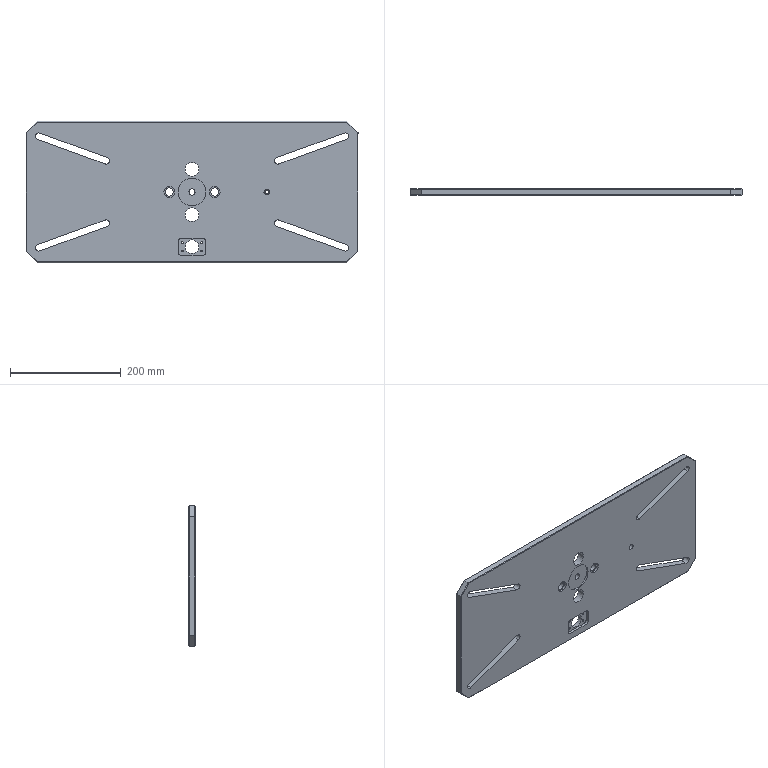Component | SolidWorks | MA060.03.03-01-1 | 1 solid | 89 faces | volume 1708847 mm3 | cylinder 46 | plane 43 | commonest cylinder face diameters 12 x12 3.3 x8 10 x6 25 x6 19.5 x4 15 x4 5.5 x2 11 x2 | material AL5052